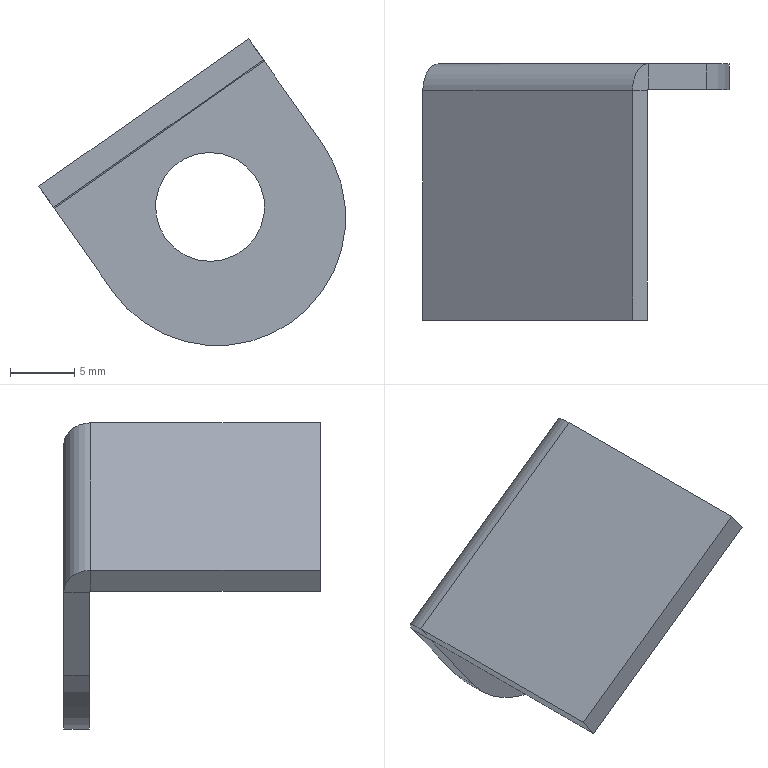Component | SolidWorks | FrontDoorLockHoleWeld-2_LockRodBracket-1 | 1 solid | 17 faces | box 23.93 x 20 x 23.93 mm | volume 1302 mm3 | plane 11 | cylinder 6 | commonest cylinder face diameters 8.5 x2 20 x2 4.2 x1 0.2 x1
STEP:
#1=CARTESIAN_POINT('',(-12.677,28.979,84.635));
#2=VERTEX_POINT('',#1);
#3=CARTESIAN_POINT('',(-12.404,28.979,84.827));
#4=VERTEX_POINT('',#3);
#5=CARTESIAN_POINT('',(-12.54,28.979,84.731));
#6=DIRECTION('',(-0.,1.,-0.));
#7=DIRECTION('',(0.818,0.,0.5751));
#8=AXIS2_PLACEMENT_3D('',#5,#6,#7);
#9=CIRCLE('',#8,0.1673);
#10=EDGE_CURVE('',#2,#4,#9,.T.);
#11=ORIENTED_EDGE('',*,*,#10,.F.);
#12=CARTESIAN_POINT('',(-12.677,29.058,84.635));
#13=VERTEX_POINT('',#12);
#14=CARTESIAN_POINT('',(-12.677,28.664,84.635));
#15=DIRECTION('',(-0.,1.,-0.));
#16=VECTOR('',#15,39.37);
#17=LINE('',#14,#16);
#18=EDGE_CURVE('',#2,#13,#17,.T.);
#19=ORIENTED_EDGE('',*,*,#18,.T.);
#20=CARTESIAN_POINT('',(-12.404,29.058,84.827));
#21=VERTEX_POINT('',#20);
#22=CARTESIAN_POINT('',(-12.54,29.058,84.731));
#23=DIRECTION('',(-0.,1.,-0.));
#24=DIRECTION('',(0.818,0.,0.5751));
#25=AXIS2_PLACEMENT_3D('',#22,#23,#24);
#26=CIRCLE('',#25,0.1673);
#27=EDGE_CURVE('',#13,#21,#26,.T.);
#28=ORIENTED_EDGE('',*,*,#27,.T.);
#29=CARTESIAN_POINT('',(-12.404,28.664,84.827));
#30=DIRECTION('',(-0.,1.,-0.));
#31=VECTOR('',#30,39.37);
#32=LINE('',#29,#31);
#33=EDGE_CURVE('',#4,#21,#32,.T.);
#34=ORIENTED_EDGE('',*,*,#33,.F.);
#35=EDGE_LOOP('',(#11,#19,#28,#34));
#36=FACE_OUTER_BOUND('',#35,.T.);
#37=CARTESIAN_POINT('',(-12.54,28.664,84.731));
#38=DIRECTION('',(-0.,1.,-0.));
#39=DIRECTION('',(0.818,0.,0.5751));
#40=AXIS2_PLACEMENT_3D('',#37,#38,#39);
#41=CYLINDRICAL_SURFACE('',#40,0.1673);
#42=ADVANCED_FACE('',(#36),#41,.F.);
#43=CARTESIAN_POINT('',(-12.84,29.058,84.472));
#44=VERTEX_POINT('',#43);
#45=CARTESIAN_POINT('',(-13.019,29.058,84.727));
#46=VERTEX_POINT('',#45);
#47=CARTESIAN_POINT('',(-12.613,29.058,84.15));
#48=DIRECTION('',(-0.5751,-0.,0.818));
#49=VECTOR('',#48,39.37);
#50=LINE('',#47,#49);
#51=EDGE_CURVE('',#44,#46,#50,.T.);
#52=ORIENTED_EDGE('',*,*,#51,.F.);
#53=CARTESIAN_POINT('',(-12.84,28.979,84.472));
#54=VERTEX_POINT('',#53);
#55=CARTESIAN_POINT('',(-12.84,28.979,84.472));
#56=DIRECTION('',(0.,-1.,0.));
#57=VECTOR('',#56,39.37);
#58=LINE('',#55,#57);
#59=EDGE_CURVE('',#44,#54,#58,.T.);
#60=ORIENTED_EDGE('',*,*,#59,.T.);
#61=CARTESIAN_POINT('',(-13.019,28.979,84.727));
#62=VERTEX_POINT('',#61);
#63=CARTESIAN_POINT('',(-12.613,28.979,84.15));
#64=DIRECTION('',(-0.5751,-0.,0.818));
#65=VECTOR('',#64,39.37);
#66=LINE('',#63,#65);
#67=EDGE_CURVE('',#54,#62,#66,.T.);
#68=ORIENTED_EDGE('',*,*,#67,.T.);
#69=CARTESIAN_POINT('',(-13.019,28.979,84.727));
#70=DIRECTION('',(-0.,1.,-0.));
#71=VECTOR('',#70,39.37);
#72=LINE('',#69,#71);
#73=EDGE_CURVE('',#62,#46,#72,.T.);
#74=ORIENTED_EDGE('',*,*,#73,.T.);
#75=EDGE_LOOP('',(#52,#60,#68,#74));
#76=FACE_OUTER_BOUND('',#75,.T.);
#77=CARTESIAN_POINT('',(-12.613,28.979,84.15));
#78=DIRECTION('',(-0.818,-0.,-0.5751));
#79=DIRECTION('',(-0.5751,-0.,0.818));
#80=AXIS2_PLACEMENT_3D('',#77,#78,#79);
#81=PLANE('',#80);
#82=ADVANCED_FACE('',(#76),#81,.T.);
#83=CARTESIAN_POINT('',(-12.54,28.979,84.731));
#84=DIRECTION('',(-0.,1.,-0.));
#85=DIRECTION('',(0.818,0.,0.5751));
#86=AXIS2_PLACEMENT_3D('',#83,#84,#85);
#87=CIRCLE('',#86,0.1673);
#88=EDGE_CURVE('',#4,#2,#87,.T.);
#89=ORIENTED_EDGE('',*,*,#88,.T.);
#90=ORIENTED_EDGE('',*,*,#10,.T.);
#91=EDGE_LOOP('',(#89,#90));
#92=FACE_BOUND('',#91,.T.);
#93=ORIENTED_EDGE('',*,*,#67,.F.);
#94=CARTESIAN_POINT('',(-12.291,28.979,84.377));
#95=VERTEX_POINT('',#94);
#96=CARTESIAN_POINT('',(-12.518,28.979,84.699));
#97=DIRECTION('',(0.,-1.,0.));
#98=DIRECTION('',(0.818,0.,0.5751));
#99=AXIS2_PLACEMENT_3D('',#96,#97,#98);
#100=CIRCLE('',#99,0.3937);
#101=EDGE_CURVE('',#54,#95,#100,.T.);
#102=ORIENTED_EDGE('',*,*,#101,.T.);
#103=CARTESIAN_POINT('',(-12.196,28.979,84.925));
#104=VERTEX_POINT('',#103);
#105=CARTESIAN_POINT('',(-12.518,28.979,84.699));
#106=DIRECTION('',(0.,-1.,0.));
#107=DIRECTION('',(0.818,0.,0.5751));
#108=AXIS2_PLACEMENT_3D('',#105,#106,#107);
#109=CIRCLE('',#108,0.3937);
#110=EDGE_CURVE('',#95,#104,#109,.T.);
#111=ORIENTED_EDGE('',*,*,#110,.T.);
#112=CARTESIAN_POINT('',(-12.375,28.979,85.18));
#113=VERTEX_POINT('',#112);
#114=CARTESIAN_POINT('',(-11.969,28.979,84.603));
#115=DIRECTION('',(0.5751,0.,-0.818));
#116=VECTOR('',#115,39.37);
#117=LINE('',#114,#116);
#118=EDGE_CURVE('',#113,#104,#117,.T.);
#119=ORIENTED_EDGE('',*,*,#118,.F.);
#120=CARTESIAN_POINT('',(-13.019,28.979,84.727));
#121=DIRECTION('',(0.818,0.,0.5751));
#122=VECTOR('',#121,39.37);
#123=LINE('',#120,#122);
#124=EDGE_CURVE('',#62,#113,#123,.T.);
#125=ORIENTED_EDGE('',*,*,#124,.F.);
#126=EDGE_LOOP('',(#93,#102,#111,#119,#125));
#127=FACE_OUTER_BOUND('',#126,.T.);
#128=CARTESIAN_POINT('',(-13.352,28.979,87.115));
#129=DIRECTION('',(-0.,1.,-0.));
#130=DIRECTION('',(0.818,0.,0.5751));
#131=AXIS2_PLACEMENT_3D('',#128,#129,#130);
#132=PLANE('',#131);
#133=ADVANCED_FACE('',(#92,#127),#132,.F.);
#134=CARTESIAN_POINT('',(-12.54,29.058,84.731));
#135=DIRECTION('',(-0.,1.,-0.));
#136=DIRECTION('',(0.818,0.,0.5751));
#137=AXIS2_PLACEMENT_3D('',#134,#135,#136);
#138=CIRCLE('',#137,0.1673);
#139=EDGE_CURVE('',#21,#13,#138,.T.);
#140=ORIENTED_EDGE('',*,*,#139,.F.);
#141=ORIENTED_EDGE('',*,*,#27,.F.);
#142=EDGE_LOOP('',(#140,#141));
#143=FACE_BOUND('',#142,.T.);
#144=CARTESIAN_POINT('',(-12.196,29.058,84.925));
#145=VERTEX_POINT('',#144);
#146=CARTESIAN_POINT('',(-12.291,29.058,84.377));
#147=VERTEX_POINT('',#146);
#148=CARTESIAN_POINT('',(-12.518,29.058,84.699));
#149=DIRECTION('',(-0.,1.,-0.));
#150=DIRECTION('',(0.818,0.,0.5751));
#151=AXIS2_PLACEMENT_3D('',#148,#149,#150);
#152=CIRCLE('',#151,0.3937);
#153=EDGE_CURVE('',#145,#147,#152,.T.);
#154=ORIENTED_EDGE('',*,*,#153,.T.);
#155=CARTESIAN_POINT('',(-12.518,29.058,84.699));
#156=DIRECTION('',(-0.,1.,-0.));
#157=DIRECTION('',(0.818,0.,0.5751));
#158=AXIS2_PLACEMENT_3D('',#155,#156,#157);
#159=CIRCLE('',#158,0.3937);
#160=EDGE_CURVE('',#147,#44,#159,.T.);
#161=ORIENTED_EDGE('',*,*,#160,.T.);
#162=ORIENTED_EDGE('',*,*,#51,.T.);
#163=CARTESIAN_POINT('',(-12.375,29.058,85.18));
#164=VERTEX_POINT('',#163);
#165=CARTESIAN_POINT('',(-13.019,29.058,84.727));
#166=DIRECTION('',(0.818,0.,0.5751));
#167=VECTOR('',#166,39.37);
#168=LINE('',#165,#167);
#169=EDGE_CURVE('',#46,#164,#168,.T.);
#170=ORIENTED_EDGE('',*,*,#169,.T.);
#171=CARTESIAN_POINT('',(-11.969,29.058,84.603));
#172=DIRECTION('',(0.5751,0.,-0.818));
#173=VECTOR('',#172,39.37);
#174=LINE('',#171,#173);
#175=EDGE_CURVE('',#164,#145,#174,.T.);
#176=ORIENTED_EDGE('',*,*,#175,.T.);
#177=EDGE_LOOP('',(#154,#161,#162,#170,#176));
#178=FACE_OUTER_BOUND('',#177,.T.);
#179=CARTESIAN_POINT('',(-13.352,29.058,87.115));
#180=DIRECTION('',(-0.,1.,-0.));
#181=DIRECTION('',(0.818,0.,0.5751));
#182=AXIS2_PLACEMENT_3D('',#179,#180,#181);
#183=PLANE('',#182);
#184=ADVANCED_FACE('',(#143,#178),#183,.T.);
#185=ORIENTED_EDGE('',*,*,#118,.T.);
#186=CARTESIAN_POINT('',(-12.196,28.979,84.925));
#187=DIRECTION('',(-0.,1.,-0.));
#188=VECTOR('',#187,39.37);
#189=LINE('',#186,#188);
#190=EDGE_CURVE('',#104,#145,#189,.T.);
#191=ORIENTED_EDGE('',*,*,#190,.T.);
#192=ORIENTED_EDGE('',*,*,#175,.F.);
#193=CARTESIAN_POINT('',(-12.375,28.979,85.18));
#194=DIRECTION('',(-0.,1.,-0.));
#195=VECTOR('',#194,39.37);
#196=LINE('',#193,#195);
#197=EDGE_CURVE('',#113,#164,#196,.T.);
#198=ORIENTED_EDGE('',*,*,#197,.F.);
#199=EDGE_LOOP('',(#185,#191,#192,#198));
#200=FACE_OUTER_BOUND('',#199,.T.);
#201=CARTESIAN_POINT('',(-11.969,28.979,84.603));
#202=DIRECTION('',(0.818,0.,0.5751));
#203=DIRECTION('',(0.5751,0.,-0.818));
#204=AXIS2_PLACEMENT_3D('',#201,#202,#203);
#205=PLANE('',#204);
#206=ADVANCED_FACE('',(#200),#205,.T.);
#207=CARTESIAN_POINT('',(-12.377,28.975,85.183));
#208=VERTEX_POINT('',#207);
#209=CARTESIAN_POINT('',(-12.422,28.975,85.247));
#210=VERTEX_POINT('',#209);
#211=CARTESIAN_POINT('',(-12.422,28.975,85.247));
#212=DIRECTION('',(-0.5751,0.,0.818));
#213=VECTOR('',#212,39.37);
#214=LINE('',#211,#213);
#215=EDGE_CURVE('',#208,#210,#214,.T.);
#216=ORIENTED_EDGE('',*,*,#215,.F.);
#217=CARTESIAN_POINT('',(-12.375,28.975,85.18));
#218=DIRECTION('',(0.818,0.,0.5751));
#219=DIRECTION('',(0.,1.,0.));
#220=AXIS2_PLACEMENT_3D('',#217,#218,#219);
#221=CIRCLE('',#220,0.003937);
#222=EDGE_CURVE('',#113,#208,#221,.T.);
#223=ORIENTED_EDGE('',*,*,#222,.F.);
#224=ORIENTED_EDGE('',*,*,#197,.T.);
#225=CARTESIAN_POINT('',(-12.375,28.975,85.18));
#226=DIRECTION('',(0.818,0.,0.5751));
#227=DIRECTION('',(0.,1.,0.));
#228=AXIS2_PLACEMENT_3D('',#225,#226,#227);
#229=CIRCLE('',#228,0.08268);
#230=EDGE_CURVE('',#164,#210,#229,.T.);
#231=ORIENTED_EDGE('',*,*,#230,.T.);
#232=EDGE_LOOP('',(#216,#223,#224,#231));
#233=FACE_OUTER_BOUND('',#232,.T.);
#234=CARTESIAN_POINT('',(-12.375,28.975,85.18));
#235=DIRECTION('',(0.818,0.,0.5751));
#236=DIRECTION('',(0.,-1.,0.));
#237=AXIS2_PLACEMENT_3D('',#234,#235,#236);
#238=PLANE('',#237);
#239=ADVANCED_FACE('',(#233),#238,.T.);
#240=CARTESIAN_POINT('',(-13.021,28.975,84.73));
#241=VERTEX_POINT('',#240);
#242=CARTESIAN_POINT('',(-13.019,28.975,84.727));
#243=DIRECTION('',(-0.818,-0.,-0.5751));
#244=DIRECTION('',(0.,1.,0.));
#245=AXIS2_PLACEMENT_3D('',#242,#243,#244);
#246=CIRCLE('',#245,0.003937);
#247=EDGE_CURVE('',#241,#62,#246,.T.);
#248=ORIENTED_EDGE('',*,*,#247,.F.);
#249=CARTESIAN_POINT('',(-13.066,28.975,84.794));
#250=VERTEX_POINT('',#249);
#251=CARTESIAN_POINT('',(-13.021,28.975,84.73));
#252=DIRECTION('',(-0.5751,0.,0.818));
#253=VECTOR('',#252,39.37);
#254=LINE('',#251,#253);
#255=EDGE_CURVE('',#241,#250,#254,.T.);
#256=ORIENTED_EDGE('',*,*,#255,.T.);
#257=CARTESIAN_POINT('',(-13.019,28.975,84.727));
#258=DIRECTION('',(-0.818,-0.,-0.5751));
#259=DIRECTION('',(0.,1.,0.));
#260=AXIS2_PLACEMENT_3D('',#257,#258,#259);
#261=CIRCLE('',#260,0.08268);
#262=EDGE_CURVE('',#250,#46,#261,.T.);
#263=ORIENTED_EDGE('',*,*,#262,.T.);
#264=ORIENTED_EDGE('',*,*,#73,.F.);
#265=EDGE_LOOP('',(#248,#256,#263,#264));
#266=FACE_OUTER_BOUND('',#265,.T.);
#267=CARTESIAN_POINT('',(-13.019,28.975,84.727));
#268=DIRECTION('',(0.818,0.,0.5751));
#269=DIRECTION('',(0.,-1.,0.));
#270=AXIS2_PLACEMENT_3D('',#267,#268,#269);
#271=PLANE('',#270);
#272=ADVANCED_FACE('',(#266),#271,.F.);
#273=ORIENTED_EDGE('',*,*,#169,.F.);
#274=ORIENTED_EDGE('',*,*,#262,.F.);
#275=CARTESIAN_POINT('',(-12.166,28.975,85.427));
#276=DIRECTION('',(-0.818,-0.,-0.5751));
#277=VECTOR('',#276,39.37);
#278=LINE('',#275,#277);
#279=EDGE_CURVE('',#210,#250,#278,.T.);
#280=ORIENTED_EDGE('',*,*,#279,.F.);
#281=ORIENTED_EDGE('',*,*,#230,.F.);
#282=EDGE_LOOP('',(#273,#274,#280,#281));
#283=FACE_OUTER_BOUND('',#282,.T.);
#284=CARTESIAN_POINT('',(-13.019,28.975,84.727));
#285=DIRECTION('',(-0.818,-0.,-0.5751));
#286=DIRECTION('',(-0.5751,0.,0.818));
#287=AXIS2_PLACEMENT_3D('',#284,#285,#286);
#288=CYLINDRICAL_SURFACE('',#287,0.08268);
#289=ADVANCED_FACE('',(#283),#288,.T.);
#290=ORIENTED_EDGE('',*,*,#124,.T.);
#291=ORIENTED_EDGE('',*,*,#222,.T.);
#292=CARTESIAN_POINT('',(-12.377,28.975,85.183));
#293=DIRECTION('',(-0.818,-0.,-0.5751));
#294=VECTOR('',#293,39.37);
#295=LINE('',#292,#294);
#296=EDGE_CURVE('',#208,#241,#295,.T.);
#297=ORIENTED_EDGE('',*,*,#296,.T.);
#298=ORIENTED_EDGE('',*,*,#247,.T.);
#299=EDGE_LOOP('',(#290,#291,#297,#298));
#300=FACE_OUTER_BOUND('',#299,.T.);
#301=CARTESIAN_POINT('',(-13.019,28.975,84.727));
#302=DIRECTION('',(-0.818,-0.,-0.5751));
#303=DIRECTION('',(-0.5751,0.,0.818));
#304=AXIS2_PLACEMENT_3D('',#301,#302,#303);
#305=CYLINDRICAL_SURFACE('',#304,0.003937);
#306=ADVANCED_FACE('',(#300),#305,.F.);
#307=CARTESIAN_POINT('',(-13.066,28.271,84.794));
#308=VERTEX_POINT('',#307);
#309=CARTESIAN_POINT('',(-13.066,28.979,84.794));
#310=DIRECTION('',(0.,1.,-0.));
#311=VECTOR('',#310,39.37);
#312=LINE('',#309,#311);
#313=EDGE_CURVE('',#308,#250,#312,.T.);
#314=ORIENTED_EDGE('',*,*,#313,.T.);
#315=ORIENTED_EDGE('',*,*,#255,.F.);
#316=CARTESIAN_POINT('',(-13.021,28.271,84.73));
#317=VERTEX_POINT('',#316);
#318=CARTESIAN_POINT('',(-13.021,29.058,84.73));
#319=DIRECTION('',(0.,1.,-0.));
#320=VECTOR('',#319,39.37);
#321=LINE('',#318,#320);
#322=EDGE_CURVE('',#317,#241,#321,.T.);
#323=ORIENTED_EDGE('',*,*,#322,.F.);
#324=CARTESIAN_POINT('',(-13.066,28.271,84.794));
#325=DIRECTION('',(0.5751,-0.,-0.818));
#326=VECTOR('',#325,39.37);
#327=LINE('',#324,#326);
#328=EDGE_CURVE('',#308,#317,#327,.T.);
#329=ORIENTED_EDGE('',*,*,#328,.F.);
#330=EDGE_LOOP('',(#314,#315,#323,#329));
#331=FACE_OUTER_BOUND('',#330,.T.);
#332=CARTESIAN_POINT('',(-13.066,28.979,84.794));
#333=DIRECTION('',(-0.818,-0.,-0.5751));
#334=DIRECTION('',(-0.,1.,-0.));
#335=AXIS2_PLACEMENT_3D('',#332,#333,#334);
#336=PLANE('',#335);
#337=ADVANCED_FACE('',(#331),#336,.T.);
#338=CARTESIAN_POINT('',(-12.377,28.271,85.183));
#339=VERTEX_POINT('',#338);
#340=CARTESIAN_POINT('',(-12.377,29.058,85.183));
#341=DIRECTION('',(-0.,-1.,0.));
#342=VECTOR('',#341,39.37);
#343=LINE('',#340,#342);
#344=EDGE_CURVE('',#208,#339,#343,.T.);
#345=ORIENTED_EDGE('',*,*,#344,.F.);
#346=ORIENTED_EDGE('',*,*,#215,.T.);
#347=CARTESIAN_POINT('',(-12.422,28.271,85.247));
#348=VERTEX_POINT('',#347);
#349=CARTESIAN_POINT('',(-12.422,28.271,85.247));
#350=DIRECTION('',(-0.,-1.,0.));
#351=VECTOR('',#350,39.37);
#352=LINE('',#349,#351);
#353=EDGE_CURVE('',#210,#348,#352,.T.);
#354=ORIENTED_EDGE('',*,*,#353,.T.);
#355=CARTESIAN_POINT('',(-12.422,28.271,85.247));
#356=DIRECTION('',(0.5751,-0.,-0.818));
#357=VECTOR('',#356,39.37);
#358=LINE('',#355,#357);
#359=EDGE_CURVE('',#348,#339,#358,.T.);
#360=ORIENTED_EDGE('',*,*,#359,.T.);
#361=EDGE_LOOP('',(#345,#346,#354,#360));
#362=FACE_OUTER_BOUND('',#361,.T.);
#363=CARTESIAN_POINT('',(-12.422,28.271,85.247));
#364=DIRECTION('',(0.818,0.,0.5751));
#365=DIRECTION('',(0.,-1.,0.));
#366=AXIS2_PLACEMENT_3D('',#363,#364,#365);
#367=PLANE('',#366);
#368=ADVANCED_FACE('',(#362),#367,.T.);
#369=ORIENTED_EDGE('',*,*,#353,.F.);
#370=ORIENTED_EDGE('',*,*,#279,.T.);
#371=ORIENTED_EDGE('',*,*,#313,.F.);
#372=CARTESIAN_POINT('',(-13.066,28.271,84.794));
#373=DIRECTION('',(-0.818,-0.,-0.5751));
#374=VECTOR('',#373,39.37);
#375=LINE('',#372,#374);
#376=EDGE_CURVE('',#348,#308,#375,.T.);
#377=ORIENTED_EDGE('',*,*,#376,.F.);
#378=EDGE_LOOP('',(#369,#370,#371,#377));
#379=FACE_OUTER_BOUND('',#378,.T.);
#380=CARTESIAN_POINT('',(-12.166,29.058,85.427));
#381=DIRECTION('',(-0.5751,0.,0.818));
#382=DIRECTION('',(-0.,-1.,0.));
#383=AXIS2_PLACEMENT_3D('',#380,#381,#382);
#384=PLANE('',#383);
#385=ADVANCED_FACE('',(#379),#384,.T.);
#386=ORIENTED_EDGE('',*,*,#296,.F.);
#387=ORIENTED_EDGE('',*,*,#344,.T.);
#388=CARTESIAN_POINT('',(-12.121,28.271,85.363));
#389=DIRECTION('',(-0.818,-0.,-0.5751));
#390=VECTOR('',#389,39.37);
#391=LINE('',#388,#390);
#392=EDGE_CURVE('',#339,#317,#391,.T.);
#393=ORIENTED_EDGE('',*,*,#392,.T.);
#394=ORIENTED_EDGE('',*,*,#322,.T.);
#395=EDGE_LOOP('',(#386,#387,#393,#394));
#396=FACE_OUTER_BOUND('',#395,.T.);
#397=CARTESIAN_POINT('',(-12.121,29.058,85.363));
#398=DIRECTION('',(-0.5751,0.,0.818));
#399=DIRECTION('',(-0.,-1.,0.));
#400=AXIS2_PLACEMENT_3D('',#397,#398,#399);
#401=PLANE('',#400);
#402=ADVANCED_FACE('',(#396),#401,.F.);
#403=ORIENTED_EDGE('',*,*,#392,.F.);
#404=ORIENTED_EDGE('',*,*,#359,.F.);
#405=ORIENTED_EDGE('',*,*,#376,.T.);
#406=ORIENTED_EDGE('',*,*,#328,.T.);
#407=EDGE_LOOP('',(#403,#404,#405,#406));
#408=FACE_OUTER_BOUND('',#407,.T.);
#409=CARTESIAN_POINT('',(-13.066,28.271,84.794));
#410=DIRECTION('',(-0.,-1.,0.));
#411=DIRECTION('',(0.5751,-0.,-0.818));
#412=AXIS2_PLACEMENT_3D('',#409,#410,#411);
#413=PLANE('',#412);
#414=ADVANCED_FACE('',(#408),#413,.T.);
#415=ORIENTED_EDGE('',*,*,#18,.F.);
#416=ORIENTED_EDGE('',*,*,#88,.F.);
#417=ORIENTED_EDGE('',*,*,#33,.T.);
#418=ORIENTED_EDGE('',*,*,#139,.T.);
#419=EDGE_LOOP('',(#415,#416,#417,#418));
#420=FACE_OUTER_BOUND('',#419,.T.);
#421=CARTESIAN_POINT('',(-12.54,28.664,84.731));
#422=DIRECTION('',(-0.,1.,-0.));
#423=DIRECTION('',(0.818,0.,0.5751));
#424=AXIS2_PLACEMENT_3D('',#421,#422,#423);
#425=CYLINDRICAL_SURFACE('',#424,0.1673);
#426=ADVANCED_FACE('',(#420),#425,.F.);
#427=ORIENTED_EDGE('',*,*,#190,.F.);
#428=ORIENTED_EDGE('',*,*,#110,.F.);
#429=CARTESIAN_POINT('',(-12.291,28.979,84.377));
#430=DIRECTION('',(0.,-1.,0.));
#431=VECTOR('',#430,39.37);
#432=LINE('',#429,#431);
#433=EDGE_CURVE('',#147,#95,#432,.T.);
#434=ORIENTED_EDGE('',*,*,#433,.F.);
#435=ORIENTED_EDGE('',*,*,#153,.F.);
#436=EDGE_LOOP('',(#427,#428,#434,#435));
#437=FACE_OUTER_BOUND('',#436,.T.);
#438=CARTESIAN_POINT('',(-12.518,28.979,84.699));
#439=DIRECTION('',(-0.,1.,-0.));
#440=DIRECTION('',(0.818,0.,0.5751));
#441=AXIS2_PLACEMENT_3D('',#438,#439,#440);
#442=CYLINDRICAL_SURFACE('',#441,0.3937);
#443=ADVANCED_FACE('',(#437),#442,.T.);
#444=ORIENTED_EDGE('',*,*,#101,.F.);
#445=ORIENTED_EDGE('',*,*,#59,.F.);
#446=ORIENTED_EDGE('',*,*,#160,.F.);
#447=ORIENTED_EDGE('',*,*,#433,.T.);
#448=EDGE_LOOP('',(#444,#445,#446,#447));
#449=FACE_OUTER_BOUND('',#448,.T.);
#450=CARTESIAN_POINT('',(-12.518,28.979,84.699));
#451=DIRECTION('',(-0.,1.,-0.));
#452=DIRECTION('',(0.818,0.,0.5751));
#453=AXIS2_PLACEMENT_3D('',#450,#451,#452);
#454=CYLINDRICAL_SURFACE('',#453,0.3937);
#455=ADVANCED_FACE('',(#449),#454,.T.);
#456=CLOSED_SHELL('',(#42,#82,#133,#184,#206,#239,#272,#289,#306,#337,#368,#385,#402,#414,#426,#443,#455));
#457=MANIFOLD_SOLID_BREP('',#456);
#458=CARTESIAN_POINT('',(0.,0.,0.));
#459=DIRECTION('',(0.,0.,1.));
#460=DIRECTION('',(1.,0.,0.));
#461=AXIS2_PLACEMENT_3D('',#458,#459,#460);
#462=(LENGTH_UNIT()NAMED_UNIT(*)SI_UNIT($,.METRE.));
#463=LENGTH_MEASURE_WITH_UNIT(LENGTH_MEASURE(0.0254),#462);
#464=DIMENSIONAL_EXPONENTS(1.,0.,0.,0.,0.,0.,0.);
#465=(CONVERSION_BASED_UNIT('',#463)LENGTH_UNIT()NAMED_UNIT(#464));
#466=UNCERTAINTY_MEASURE_WITH_UNIT(LENGTH_MEASURE(0.00001),#465,'','');
#467=(NAMED_UNIT(*)PLANE_ANGLE_UNIT()SI_UNIT($,.RADIAN.));
#468=(NAMED_UNIT(*)SI_UNIT($,.STERADIAN.)SOLID_ANGLE_UNIT());
#469=(GEOMETRIC_REPRESENTATION_CONTEXT(3)GLOBAL_UNCERTAINTY_ASSIGNED_CONTEXT((#466))GLOBAL_UNIT_ASSIGNED_CONTEXT((#465,#467,#468))REPRESENTATION_CONTEXT('',''));
#470=ADVANCED_BREP_SHAPE_REPRESENTATION('',(#457,#461),#469);
#471=COLOUR_RGB('',0.7922,0.8196,0.9333);
#472=FILL_AREA_STYLE_COLOUR('',#471);
#473=FILL_AREA_STYLE('',(#472));
#474=SURFACE_STYLE_FILL_AREA(#473);
#475=SURFACE_SIDE_STYLE('',(#474));
#476=SURFACE_STYLE_USAGE(.BOTH.,#475);
#477=PRESENTATION_STYLE_ASSIGNMENT((#476));
#478=STYLED_ITEM('',(#477),#457);
#479=(LENGTH_UNIT()NAMED_UNIT(*)SI_UNIT($,.METRE.));
#480=LENGTH_MEASURE_WITH_UNIT(LENGTH_MEASURE(0.0254),#479);
#481=DIMENSIONAL_EXPONENTS(1.,0.,0.,0.,0.,0.,0.);
#482=(CONVERSION_BASED_UNIT('',#480)LENGTH_UNIT()NAMED_UNIT(#481));
#483=UNCERTAINTY_MEASURE_WITH_UNIT(LENGTH_MEASURE(0.00001),#482,'','');
#484=(NAMED_UNIT(*)PLANE_ANGLE_UNIT()SI_UNIT($,.RADIAN.));
#485=(NAMED_UNIT(*)SI_UNIT($,.STERADIAN.)SOLID_ANGLE_UNIT());
#486=(GEOMETRIC_REPRESENTATION_CONTEXT(3)GLOBAL_UNCERTAINTY_ASSIGNED_CONTEXT((#483))GLOBAL_UNIT_ASSIGNED_CONTEXT((#482,#484,#485))REPRESENTATION_CONTEXT('',''));
#487=MECHANICAL_DESIGN_GEOMETRIC_PRESENTATION_REPRESENTATION('',(#478),#486);
#488=PRESENTATION_LAYER_ASSIGNMENT('','',(#478));